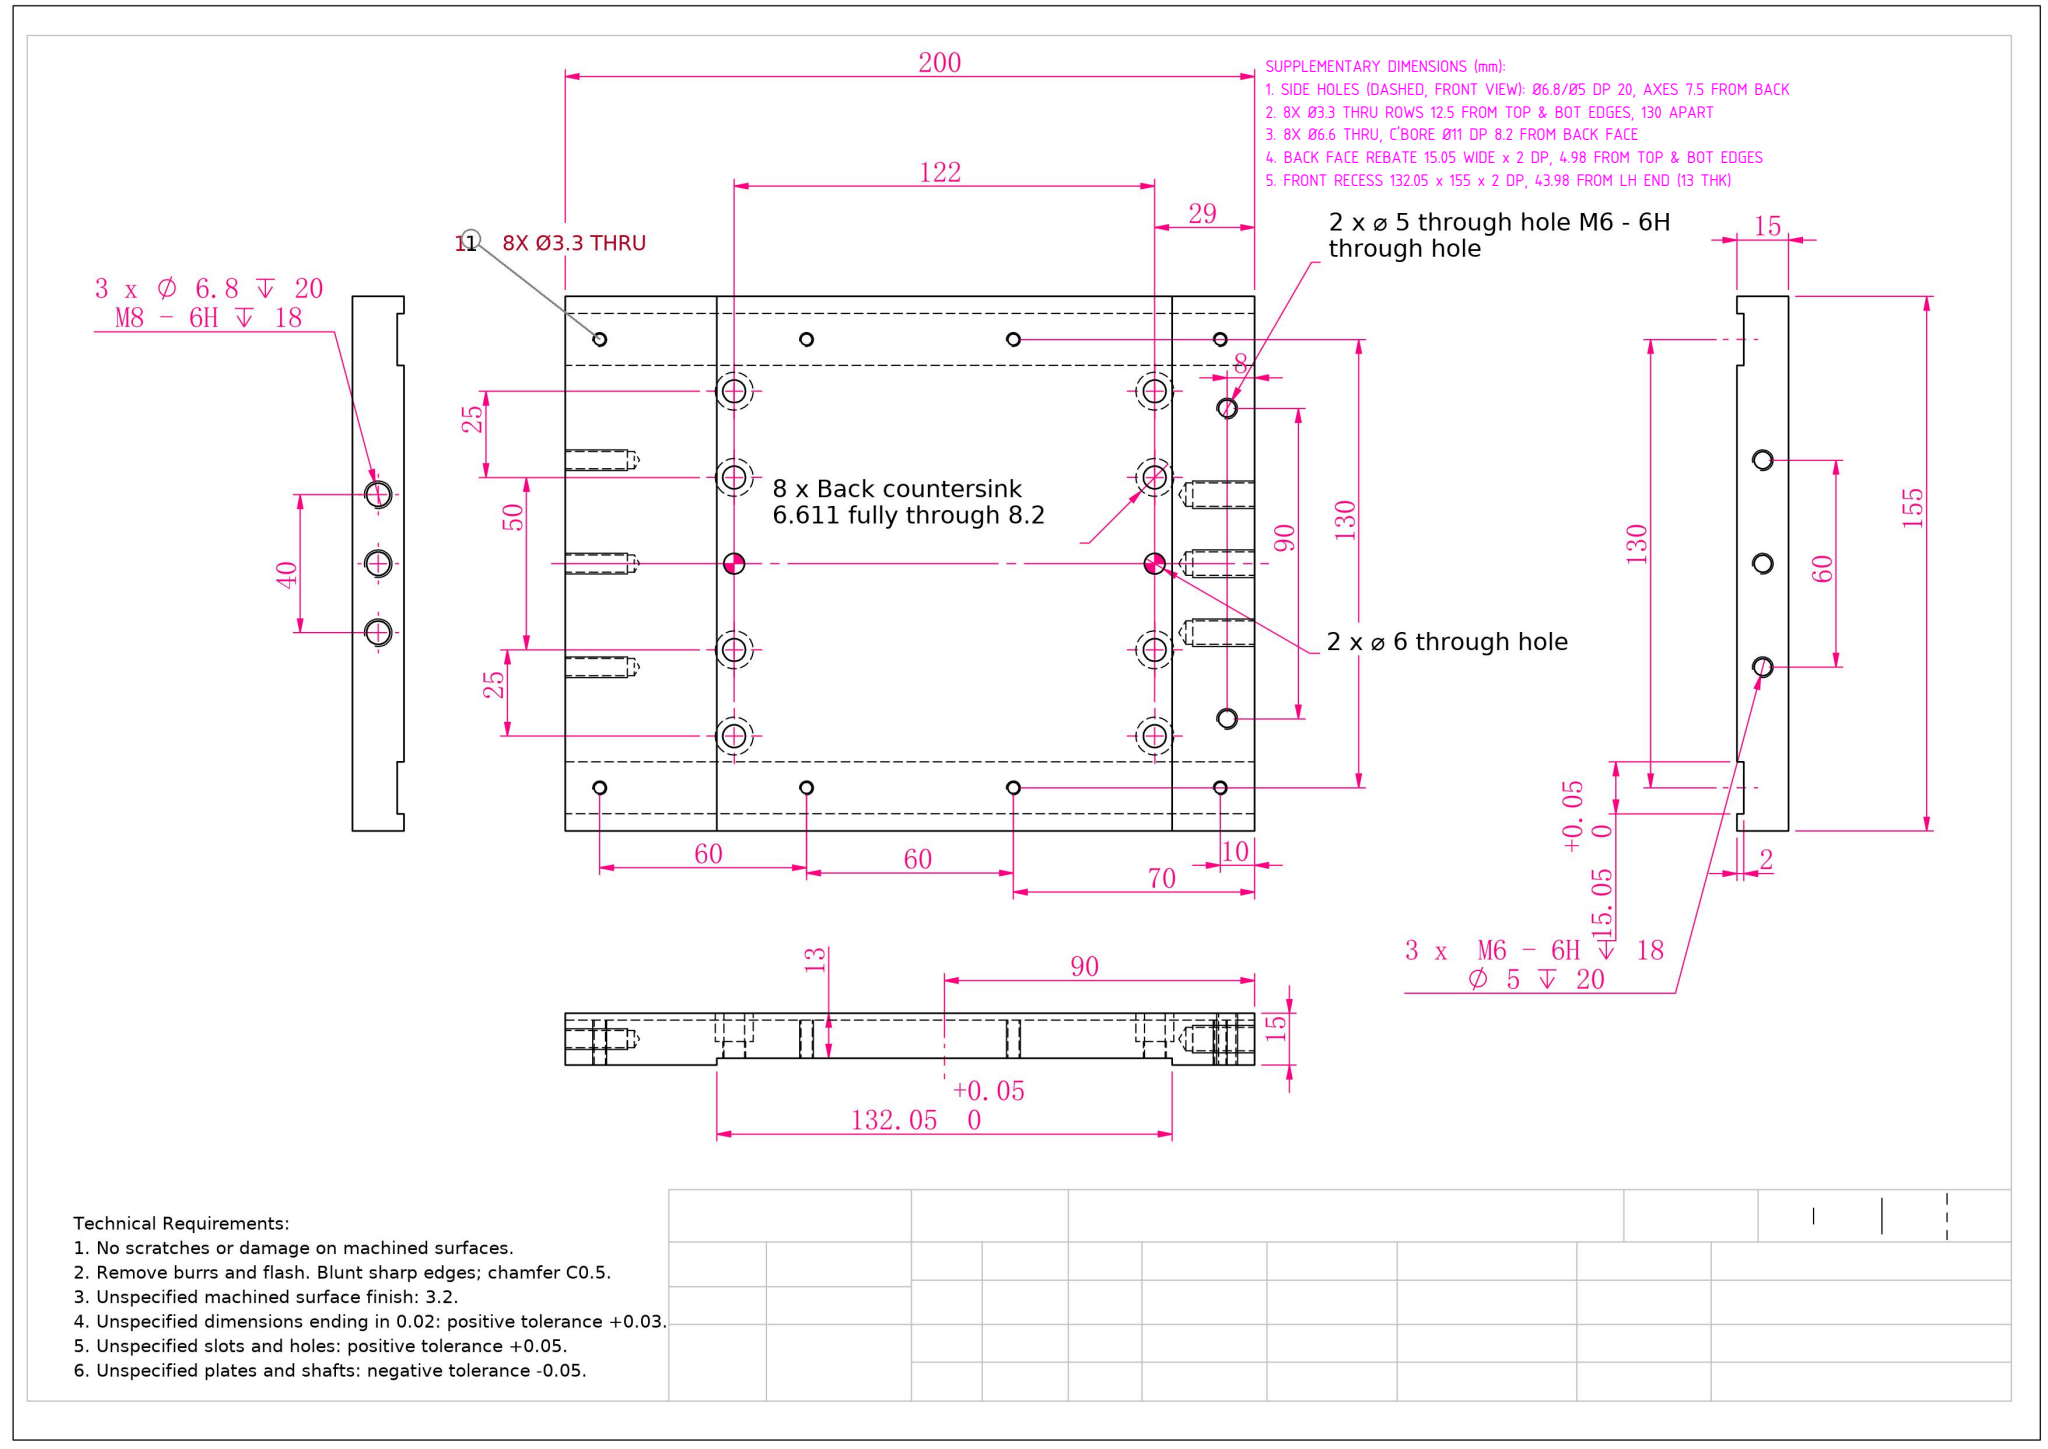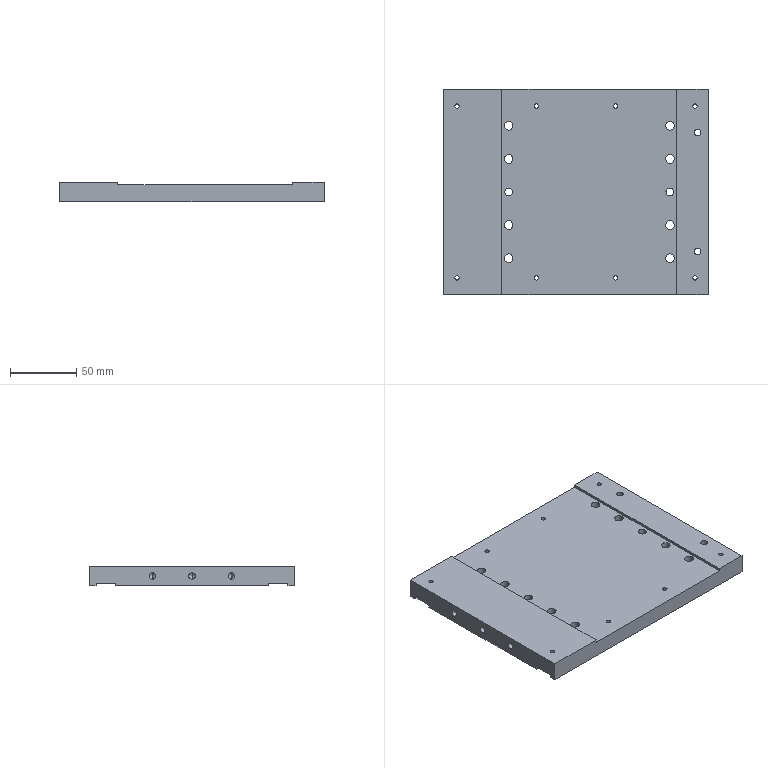Part | SolidWorks | mm | 1 solid | 106 faces | box 200 x 155 x 15 mm | volume 398871 mm3 | cylinder 68 | plane 26 | cone 12 | commonest cylinder face diameters 3.3 x16 11 x16 6.6 x16 5 x10 6.8 x6 6 x4
build123d program:
from build123d import *

# Parameters (mm, degrees)
SKETCH1_W                                       = 200
SKETCH1_H                                       = 155
BOSS_EXTRUDE1_DEPTH                             = 7.5
SKETCH2_W                                       = 132.05
SKETCH2_H                                       = 155
CUT_EXTRUDE1_DEPTH                              = 2
SKETCH10_W                                      = 230
SKETCH10_H                                      = 15.05
CUT_EXTRUDE2_DEPTH                              = 2
M6_HEX_SOCKET_HEAD_CAP_SCREW_CBORE1_D           = 6.6
M6_HEX_SOCKET_HEAD_CAP_SCREW_CBORE1_CBORE_D     = 11
M6_HEX_SOCKET_HEAD_CAP_SCREW_CBORE1_CBORE_DEPTH = 8.2
SIZE_MM_DOWEL_HOLE1_D                           = 6
M4_TAPPED_HOLE1_D                               = 3.3
M8_TAPPED_HOLE1_D                               = 6.8
M8_TAPPED_HOLE1_DEPTH                           = 20
M8_TAPPED_HOLE1_TIP                             = 2.043
M6_TAPPED_HOLE1_D                               = 5
M6_TAPPED_HOLE1_DEPTH                           = 20
M6_TAPPED_HOLE1_TIP                             = 1.502
M6_TAPPED_HOLE2_D                               = 5


with BuildPart() as part:
    # Sketch1 → Boss-Extrude1 (new, symmetric)
    with BuildSketch(Plane.XY):
        Rectangle(SKETCH1_W, SKETCH1_H)
    extrude(amount=BOSS_EXTRUDE1_DEPTH, both=True)

    # Sketch2 → Cut-Extrude1 (cut)
    with BuildSketch(Plane.XY.offset(7.5)):
        with Locations((10, 0)):
            Rectangle(SKETCH2_W, SKETCH2_H)
    extrude(amount=-CUT_EXTRUDE1_DEPTH, mode=Mode.SUBTRACT)

    # Sketch10 → Cut-Extrude2 (cut)
    with BuildSketch(Plane(origin=(0, 0, -7.5), x_dir=(-1, 0, 0), z_dir=(0, 0, -1))):
        with Locations((-15, 65)):
            Rectangle(SKETCH10_W, SKETCH10_H)
        with Locations((-15, -65)):
            Rectangle(SKETCH10_W, SKETCH10_H)
    extrude(amount=-CUT_EXTRUDE2_DEPTH, mode=Mode.SUBTRACT)

    # M6 Hex Socket Head Cap Screw CBORE1 (through all)
    with Locations(Plane(origin=(0, 0, -7.5), x_dir=(-1, 0, 0), z_dir=(0, 0, -1))):
        with Locations((51, 50), (51, 25), (51, -25), (51, -50), (-71, -50), (-71, -25), (-71, 25), (-71, 50)):
            CounterBoreHole(M6_HEX_SOCKET_HEAD_CAP_SCREW_CBORE1_D / 2, M6_HEX_SOCKET_HEAD_CAP_SCREW_CBORE1_CBORE_D / 2, M6_HEX_SOCKET_HEAD_CAP_SCREW_CBORE1_CBORE_DEPTH)

    # Size mm Dowel Hole1 (through all)
    with Locations(Plane(origin=(0, 0, -7.5), x_dir=(-1, 0, 0), z_dir=(0, 0, -1))):
        with Locations((51, 0), (-71, 0)):
            Hole(SIZE_MM_DOWEL_HOLE1_D / 2)

    # M4 Tapped Hole1 (through all)
    with Locations(Plane(origin=(0, 0, -7.5), x_dir=(-1, 0, 0), z_dir=(0, 0, -1))):
        with Locations((90, -65), (30, -65), (-30, -65), (-30, 65), (30, 65), (90, 65), (-90, 65), (-90, -65)):
            Hole(M4_TAPPED_HOLE1_D / 2)

    # M8 Tapped Hole1
    with Locations(Plane(origin=(100, 0, 0), x_dir=(0, 0, -1), z_dir=(1, 0, 0))):
        with Locations((0, 20), (0, 0), (0, -20)):
            Hole(M8_TAPPED_HOLE1_D / 2, depth=M8_TAPPED_HOLE1_DEPTH)
            with Locations((0, 0, -(M8_TAPPED_HOLE1_DEPTH + M8_TAPPED_HOLE1_TIP / 2))):  # 118° drill point
                Cone(0, M8_TAPPED_HOLE1_D / 2, M8_TAPPED_HOLE1_TIP, mode=Mode.SUBTRACT)

    # M6 Tapped Hole1
    with Locations(Plane.ZY.offset(100)):
        with Locations((0, -30), (0, 0), (0, 30)):
            Hole(M6_TAPPED_HOLE1_D / 2, depth=M6_TAPPED_HOLE1_DEPTH)
            with Locations((0, 0, -(M6_TAPPED_HOLE1_DEPTH + M6_TAPPED_HOLE1_TIP / 2))):  # 118° drill point
                Cone(0, M6_TAPPED_HOLE1_D / 2, M6_TAPPED_HOLE1_TIP, mode=Mode.SUBTRACT)

    # M6 Tapped Hole2 (through all)
    with Locations(Plane(origin=(0, 0, -7.5), x_dir=(-1, 0, 0), z_dir=(0, 0, -1))):
        with Locations((-92, -45), (-92, 45)):
            Hole(M6_TAPPED_HOLE2_D / 2)


solid = part.part